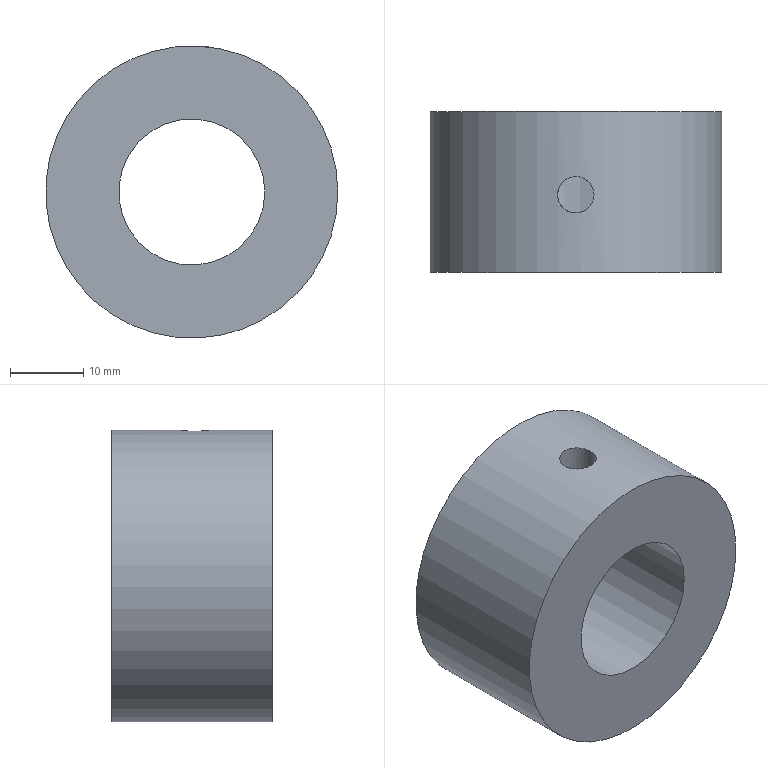Component | NX | BUSHING_5 | 1 solid | 5 faces | box 40 x 22 x 40 mm | volume 20537 mm3 | cylinder 3 | plane 2 | commonest cylinder face diameters 40 x1 20 x1 5 x1
STEP:
#1=CARTESIAN_POINT('',(0.,0.,0.));
#2=DIRECTION('',(0.,0.,1.));
#3=DIRECTION('',(1.,0.,0.));
#4=AXIS2_PLACEMENT_3D('',#1,#2,#3);
#5=CARTESIAN_POINT('',(1454.254,1145.,813.574));
#6=VERTEX_POINT('',#5);
#7=CARTESIAN_POINT('',(1434.254,1145.,813.574));
#8=DIRECTION('',(0.,1.,0.));
#9=DIRECTION('',(1.,0.,0.));
#10=AXIS2_PLACEMENT_3D('',#7,#8,#9);
#11=CIRCLE('',#10,20.);
#12=CARTESIAN_POINT('',(1434.254,1145.,813.574));
#13=DIRECTION('',(0.,-1.,0.));
#14=DIRECTION('',(0.,0.,-1.));
#15=AXIS2_PLACEMENT_3D('',#12,#13,#14);
#16=CYLINDRICAL_SURFACE('',#15,20.);
#17=CARTESIAN_POINT('',(7.854,0.));
#18=DIRECTION('',(-1.,0.));
#19=VECTOR('',#18,1.);
#20=LINE('',#17,#19);
#21=(GEOMETRIC_REPRESENTATION_CONTEXT(2)PARAMETRIC_REPRESENTATION_CONTEXT()REPRESENTATION_CONTEXT('',''));
#22=DEFINITIONAL_REPRESENTATION('',(#20),#21);
#23=PCURVE('',#16,#22);
#24=CARTESIAN_POINT('',(1434.254,1145.,813.574));
#25=DIRECTION('',(0.,1.,0.));
#26=DIRECTION('',(0.,0.,1.));
#27=AXIS2_PLACEMENT_3D('',#24,#25,#26);
#28=PLANE('',#27);
#29=CARTESIAN_POINT('',(0.,0.));
#30=DIRECTION('',(0.,1.));
#31=AXIS2_PLACEMENT_2D('',#29,#30);
#32=CIRCLE('',#31,20.);
#33=(GEOMETRIC_REPRESENTATION_CONTEXT(2)PARAMETRIC_REPRESENTATION_CONTEXT()REPRESENTATION_CONTEXT('',''));
#34=DEFINITIONAL_REPRESENTATION('',(#32),#33);
#35=PCURVE('',#28,#34);
#36=SURFACE_CURVE('',#11,(#23,#35),.PCURVE_S1.);
#37=EDGE_CURVE('',#6,#6,#36,.T.);
#38=ORIENTED_EDGE('',*,*,#37,.F.);
#39=CARTESIAN_POINT('',(1454.254,1123.,813.574));
#40=VERTEX_POINT('',#39);
#41=CARTESIAN_POINT('',(1454.254,1145.,813.574));
#42=CARTESIAN_POINT('',(1454.254,1123.,813.574));
#43=B_SPLINE_CURVE_WITH_KNOTS('',1,(#41,#42),.UNSPECIFIED.,.F.,.F.,(2,2),(0.,22.),.PIECEWISE_BEZIER_KNOTS.);
#44=CARTESIAN_POINT('',(7.854,0.));
#45=DIRECTION('',(0.,1.));
#46=VECTOR('',#45,1.);
#47=LINE('',#44,#46);
#48=(GEOMETRIC_REPRESENTATION_CONTEXT(2)PARAMETRIC_REPRESENTATION_CONTEXT()REPRESENTATION_CONTEXT('',''));
#49=DEFINITIONAL_REPRESENTATION('',(#47),#48);
#50=PCURVE('',#16,#49);
#51=CARTESIAN_POINT('',(1.571,0.));
#52=DIRECTION('',(0.,1.));
#53=VECTOR('',#52,1.);
#54=LINE('',#51,#53);
#55=(GEOMETRIC_REPRESENTATION_CONTEXT(2)PARAMETRIC_REPRESENTATION_CONTEXT()REPRESENTATION_CONTEXT('',''));
#56=DEFINITIONAL_REPRESENTATION('',(#54),#55);
#57=PCURVE('',#16,#56);
#58=SEAM_CURVE('',#43,(#50,#57),.PCURVE_S1.);
#59=EDGE_CURVE('',#6,#40,#58,.T.);
#60=ORIENTED_EDGE('',*,*,#59,.T.);
#61=CARTESIAN_POINT('',(1434.254,1123.,813.574));
#62=DIRECTION('',(0.,1.,0.));
#63=DIRECTION('',(1.,0.,0.));
#64=AXIS2_PLACEMENT_3D('',#61,#62,#63);
#65=CIRCLE('',#64,20.);
#66=CARTESIAN_POINT('',(7.854,22.));
#67=DIRECTION('',(-1.,0.));
#68=VECTOR('',#67,1.);
#69=LINE('',#66,#68);
#70=(GEOMETRIC_REPRESENTATION_CONTEXT(2)PARAMETRIC_REPRESENTATION_CONTEXT()REPRESENTATION_CONTEXT('',''));
#71=DEFINITIONAL_REPRESENTATION('',(#69),#70);
#72=PCURVE('',#16,#71);
#73=CARTESIAN_POINT('',(1434.254,1123.,813.574));
#74=DIRECTION('',(0.,1.,0.));
#75=DIRECTION('',(0.,0.,1.));
#76=AXIS2_PLACEMENT_3D('',#73,#74,#75);
#77=PLANE('',#76);
#78=CARTESIAN_POINT('',(0.,0.));
#79=DIRECTION('',(0.,1.));
#80=AXIS2_PLACEMENT_2D('',#78,#79);
#81=CIRCLE('',#80,20.);
#82=(GEOMETRIC_REPRESENTATION_CONTEXT(2)PARAMETRIC_REPRESENTATION_CONTEXT()REPRESENTATION_CONTEXT('',''));
#83=DEFINITIONAL_REPRESENTATION('',(#81),#82);
#84=PCURVE('',#77,#83);
#85=SURFACE_CURVE('',#65,(#72,#84),.PCURVE_S1.);
#86=EDGE_CURVE('',#40,#40,#85,.T.);
#87=ORIENTED_EDGE('',*,*,#86,.T.);
#88=ORIENTED_EDGE('',*,*,#59,.F.);
#89=EDGE_LOOP('',(#38,#60,#87,#88));
#90=FACE_BOUND('',#89,.T.);
#91=CARTESIAN_POINT('',(1436.754,1133.59,833.417));
#92=VERTEX_POINT('',#91);
#93=CARTESIAN_POINT('',(1436.754,1133.59,833.417));
#94=CARTESIAN_POINT('',(1436.754,1133.312,833.417));
#95=CARTESIAN_POINT('',(1436.706,1133.029,833.423));
#96=CARTESIAN_POINT('',(1436.615,1132.766,833.434));
#97=CARTESIAN_POINT('',(1436.523,1132.504,833.445));
#98=CARTESIAN_POINT('',(1436.385,1132.253,833.46));
#99=CARTESIAN_POINT('',(1436.212,1132.036,833.478));
#100=CARTESIAN_POINT('',(1436.038,1131.817,833.495));
#101=CARTESIAN_POINT('',(1435.824,1131.625,833.513));
#102=CARTESIAN_POINT('',(1435.588,1131.476,833.529));
#103=CARTESIAN_POINT('',(1435.351,1131.326,833.545));
#104=CARTESIAN_POINT('',(1435.084,1131.216,833.558));
#105=CARTESIAN_POINT('',(1434.811,1131.153,833.566));
#106=CARTESIAN_POINT('',(1434.539,1131.091,833.573));
#107=CARTESIAN_POINT('',(1434.252,1131.075,833.575));
#108=CARTESIAN_POINT('',(1433.974,1131.106,833.572));
#109=CARTESIAN_POINT('',(1433.698,1131.137,833.568));
#110=CARTESIAN_POINT('',(1433.424,1131.216,833.558));
#111=CARTESIAN_POINT('',(1433.173,1131.336,833.544));
#112=CARTESIAN_POINT('',(1432.923,1131.456,833.531));
#113=CARTESIAN_POINT('',(1432.689,1131.621,833.513));
#114=CARTESIAN_POINT('',(1432.492,1131.817,833.496));
#115=CARTESIAN_POINT('',(1432.293,1132.014,833.478));
#116=CARTESIAN_POINT('',(1432.126,1132.249,833.46));
#117=CARTESIAN_POINT('',(1432.004,1132.501,833.447));
#118=CARTESIAN_POINT('',(1431.882,1132.753,833.433));
#119=CARTESIAN_POINT('',(1431.802,1133.03,833.423));
#120=CARTESIAN_POINT('',(1431.77,1133.309,833.419));
#121=CARTESIAN_POINT('',(1431.739,1133.586,833.415));
#122=CARTESIAN_POINT('',(1431.754,1133.872,833.417));
#123=CARTESIAN_POINT('',(1431.816,1134.143,833.424));
#124=CARTESIAN_POINT('',(1431.878,1134.414,833.432));
#125=CARTESIAN_POINT('',(1431.986,1134.678,833.445));
#126=CARTESIAN_POINT('',(1432.133,1134.913,833.461));
#127=CARTESIAN_POINT('',(1432.28,1135.15,833.476));
#128=CARTESIAN_POINT('',(1432.47,1135.364,833.495));
#129=CARTESIAN_POINT('',(1432.688,1135.539,833.512));
#130=CARTESIAN_POINT('',(1432.906,1135.714,833.529));
#131=CARTESIAN_POINT('',(1433.158,1135.855,833.545));
#132=CARTESIAN_POINT('',(1433.423,1135.948,833.556));
#133=CARTESIAN_POINT('',(1433.687,1136.041,833.567));
#134=CARTESIAN_POINT('',(1433.97,1136.09,833.573));
#135=CARTESIAN_POINT('',(1434.25,1136.09,833.574));
#136=CARTESIAN_POINT('',(1434.528,1136.091,833.574));
#137=CARTESIAN_POINT('',(1434.81,1136.043,833.568));
#138=CARTESIAN_POINT('',(1435.073,1135.952,833.557));
#139=CARTESIAN_POINT('',(1435.336,1135.861,833.546));
#140=CARTESIAN_POINT('',(1435.586,1135.724,833.53));
#141=CARTESIAN_POINT('',(1435.804,1135.552,833.513));
#142=CARTESIAN_POINT('',(1436.023,1135.379,833.496));
#143=CARTESIAN_POINT('',(1436.215,1135.166,833.478));
#144=CARTESIAN_POINT('',(1436.365,1134.93,833.462));
#145=CARTESIAN_POINT('',(1436.515,1134.693,833.446));
#146=CARTESIAN_POINT('',(1436.627,1134.427,833.432));
#147=CARTESIAN_POINT('',(1436.69,1134.154,833.425));
#148=CARTESIAN_POINT('',(1436.732,1133.97,833.419));
#149=CARTESIAN_POINT('',(1436.754,1133.779,833.417));
#150=CARTESIAN_POINT('',(1436.754,1133.59,833.417));
#151=B_SPLINE_CURVE_WITH_KNOTS('',3,(#93,#94,#95,#96,#97,#98,#99,#100,#101,#102,#103,#104,#105,#106,#107,#108,#109,#110,#111,#112,#113,#114,#115,#116,#117,#118,#119,#120,#121,#122,#123,#124,#125,#126,#127,#128,#129,#130,#131,#132,#133,#134,#135,#136,#137,#138,#139,#140,#141,#142,#143,#144,#145,#146,#147,#148,#149,#150),.UNSPECIFIED.,.T.,.F.,(1,3,3,3,3,3,3,3,3,3,3,3,3,3,3,3,3,3,3,3,3,1),(-0.03595,0.,0.05342,0.1068,0.1605,0.2143,0.2679,0.3212,0.3746,0.4283,0.4821,0.5356,0.5888,0.6424,0.6962,0.7499,0.8032,0.8565,0.9102,0.964,1.,1.053),.UNSPECIFIED.);
#152=CARTESIAN_POINT('',(3.016,11.41));
#153=CARTESIAN_POINT('',(3.016,11.469));
#154=CARTESIAN_POINT('',(3.016,11.588));
#155=CARTESIAN_POINT('',(3.017,11.766));
#156=CARTESIAN_POINT('',(3.019,11.942));
#157=CARTESIAN_POINT('',(3.021,12.116));
#158=CARTESIAN_POINT('',(3.024,12.284));
#159=CARTESIAN_POINT('',(3.028,12.449));
#160=CARTESIAN_POINT('',(3.032,12.609));
#161=CARTESIAN_POINT('',(3.036,12.763));
#162=CARTESIAN_POINT('',(3.041,12.91));
#163=CARTESIAN_POINT('',(3.047,13.048));
#164=CARTESIAN_POINT('',(3.053,13.178));
#165=CARTESIAN_POINT('',(3.06,13.3));
#166=CARTESIAN_POINT('',(3.067,13.412));
#167=CARTESIAN_POINT('',(3.074,13.514));
#168=CARTESIAN_POINT('',(3.082,13.605));
#169=CARTESIAN_POINT('',(3.09,13.685));
#170=CARTESIAN_POINT('',(3.098,13.753));
#171=CARTESIAN_POINT('',(3.106,13.81));
#172=CARTESIAN_POINT('',(3.115,13.854));
#173=CARTESIAN_POINT('',(3.124,13.886));
#174=CARTESIAN_POINT('',(3.133,13.905));
#175=CARTESIAN_POINT('',(3.142,13.912));
#176=CARTESIAN_POINT('',(3.151,13.905));
#177=CARTESIAN_POINT('',(3.159,13.886));
#178=CARTESIAN_POINT('',(3.168,13.855));
#179=CARTESIAN_POINT('',(3.177,13.81));
#180=CARTESIAN_POINT('',(3.185,13.754));
#181=CARTESIAN_POINT('',(3.194,13.686));
#182=CARTESIAN_POINT('',(3.202,13.606));
#183=CARTESIAN_POINT('',(3.209,13.515));
#184=CARTESIAN_POINT('',(3.217,13.413));
#185=CARTESIAN_POINT('',(3.224,13.301));
#186=CARTESIAN_POINT('',(3.23,13.18));
#187=CARTESIAN_POINT('',(3.236,13.049));
#188=CARTESIAN_POINT('',(3.242,12.91));
#189=CARTESIAN_POINT('',(3.247,12.763));
#190=CARTESIAN_POINT('',(3.252,12.61));
#191=CARTESIAN_POINT('',(3.256,12.451));
#192=CARTESIAN_POINT('',(3.259,12.286));
#193=CARTESIAN_POINT('',(3.262,12.116));
#194=CARTESIAN_POINT('',(3.264,11.943));
#195=CARTESIAN_POINT('',(3.266,11.767));
#196=CARTESIAN_POINT('',(3.267,11.59));
#197=CARTESIAN_POINT('',(3.267,11.412));
#198=CARTESIAN_POINT('',(3.267,11.232));
#199=CARTESIAN_POINT('',(3.266,11.054));
#200=CARTESIAN_POINT('',(3.264,10.879));
#201=CARTESIAN_POINT('',(3.262,10.706));
#202=CARTESIAN_POINT('',(3.259,10.537));
#203=CARTESIAN_POINT('',(3.256,10.371));
#204=CARTESIAN_POINT('',(3.252,10.211));
#205=CARTESIAN_POINT('',(3.247,10.058));
#206=CARTESIAN_POINT('',(3.242,9.912));
#207=CARTESIAN_POINT('',(3.236,9.773));
#208=CARTESIAN_POINT('',(3.23,9.642));
#209=CARTESIAN_POINT('',(3.224,9.52));
#210=CARTESIAN_POINT('',(3.217,9.408));
#211=CARTESIAN_POINT('',(3.209,9.306));
#212=CARTESIAN_POINT('',(3.202,9.215));
#213=CARTESIAN_POINT('',(3.194,9.135));
#214=CARTESIAN_POINT('',(3.185,9.066));
#215=CARTESIAN_POINT('',(3.177,9.01));
#216=CARTESIAN_POINT('',(3.168,8.966));
#217=CARTESIAN_POINT('',(3.16,8.934));
#218=CARTESIAN_POINT('',(3.151,8.914));
#219=CARTESIAN_POINT('',(3.142,8.908));
#220=CARTESIAN_POINT('',(3.133,8.914));
#221=CARTESIAN_POINT('',(3.124,8.933));
#222=CARTESIAN_POINT('',(3.115,8.965));
#223=CARTESIAN_POINT('',(3.106,9.009));
#224=CARTESIAN_POINT('',(3.098,9.065));
#225=CARTESIAN_POINT('',(3.09,9.133));
#226=CARTESIAN_POINT('',(3.082,9.213));
#227=CARTESIAN_POINT('',(3.074,9.304));
#228=CARTESIAN_POINT('',(3.067,9.406));
#229=CARTESIAN_POINT('',(3.06,9.517));
#230=CARTESIAN_POINT('',(3.053,9.639));
#231=CARTESIAN_POINT('',(3.047,9.769));
#232=CARTESIAN_POINT('',(3.041,9.908));
#233=CARTESIAN_POINT('',(3.036,10.054));
#234=CARTESIAN_POINT('',(3.032,10.207));
#235=CARTESIAN_POINT('',(3.028,10.367));
#236=CARTESIAN_POINT('',(3.024,10.532));
#237=CARTESIAN_POINT('',(3.021,10.702));
#238=CARTESIAN_POINT('',(3.019,10.874));
#239=CARTESIAN_POINT('',(3.017,11.051));
#240=CARTESIAN_POINT('',(3.016,11.23));
#241=CARTESIAN_POINT('',(3.016,11.35));
#242=CARTESIAN_POINT('',(3.016,11.41));
#243=B_SPLINE_CURVE_WITH_KNOTS('',3,(#152,#153,#154,#155,#156,#157,#158,#159,#160,#161,#162,#163,#164,#165,#166,#167,#168,#169,#170,#171,#172,#173,#174,#175,#176,#177,#178,#179,#180,#181,#182,#183,#184,#185,#186,#187,#188,#189,#190,#191,#192,#193,#194,#195,#196,#197,#198,#199,#200,#201,#202,#203,#204,#205,#206,#207,#208,#209,#210,#211,#212,#213,#214,#215,#216,#217,#218,#219,#220,#221,#222,#223,#224,#225,#226,#227,#228,#229,#230,#231,#232,#233,#234,#235,#236,#237,#238,#239,#240,#241,#242),.UNSPECIFIED.,.T.,.F.,(4,1,1,1,1,1,1,1,1,1,1,1,1,1,1,1,1,1,1,1,1,1,1,1,1,1,1,1,1,1,1,1,1,1,1,1,1,1,1,1,1,1,1,1,1,1,1,1,1,1,1,1,1,1,1,1,1,1,1,1,1,1,1,1,1,1,1,1,1,1,1,1,1,1,1,1,1,1,1,1,1,1,1,1,1,1,1,1,4),(0.,0.01136,0.02273,0.03409,0.04545,0.05682,0.06818,0.07955,0.09091,0.1023,0.1136,0.125,0.1364,0.1477,0.1591,0.1705,0.1818,0.1932,0.2045,0.2159,0.2273,0.2386,0.25,0.2614,0.2727,0.2841,0.2955,0.3068,0.3182,0.3295,0.3409,0.3523,0.3636,0.375,0.3864,0.3977,0.4091,0.4205,0.4318,0.4432,0.4545,0.4659,0.4773,0.4886,0.5,0.5114,0.5227,0.5341,0.5455,0.5568,0.5682,0.5795,0.5909,0.6023,0.6136,0.625,0.6364,0.6477,0.6591,0.6705,0.6818,0.6932,0.7045,0.7159,0.7273,0.7386,0.75,0.7614,0.7727,0.7841,0.7955,0.8068,0.8182,0.8295,0.8409,0.8523,0.8636,0.875,0.8864,0.8977,0.9091,0.9205,0.9318,0.9432,0.9545,0.9659,0.9773,0.9886,1.),.QUASI_UNIFORM_KNOTS.);
#244=(GEOMETRIC_REPRESENTATION_CONTEXT(2)PARAMETRIC_REPRESENTATION_CONTEXT()REPRESENTATION_CONTEXT('',''));
#245=DEFINITIONAL_REPRESENTATION('',(#243),#244);
#246=PCURVE('',#16,#245);
#247=CARTESIAN_POINT('',(1434.254,1133.59,813.574));
#248=DIRECTION('',(-0.,0.,1.));
#249=DIRECTION('',(1.,0.,0.));
#250=AXIS2_PLACEMENT_3D('',#247,#248,#249);
#251=CYLINDRICAL_SURFACE('',#250,2.5);
#252=CARTESIAN_POINT('',(6.283,19.843));
#253=CARTESIAN_POINT('',(6.259,19.843));
#254=CARTESIAN_POINT('',(6.212,19.844));
#255=CARTESIAN_POINT('',(6.14,19.846));
#256=CARTESIAN_POINT('',(6.069,19.85));
#257=CARTESIAN_POINT('',(5.997,19.855));
#258=CARTESIAN_POINT('',(5.926,19.862));
#259=CARTESIAN_POINT('',(5.855,19.87));
#260=CARTESIAN_POINT('',(5.783,19.879));
#261=CARTESIAN_POINT('',(5.712,19.889));
#262=CARTESIAN_POINT('',(5.64,19.9));
#263=CARTESIAN_POINT('',(5.569,19.91));
#264=CARTESIAN_POINT('',(5.498,19.922));
#265=CARTESIAN_POINT('',(5.427,19.933));
#266=CARTESIAN_POINT('',(5.355,19.944));
#267=CARTESIAN_POINT('',(5.284,19.954));
#268=CARTESIAN_POINT('',(5.213,19.964));
#269=CARTESIAN_POINT('',(5.141,19.973));
#270=CARTESIAN_POINT('',(5.07,19.981));
#271=CARTESIAN_POINT('',(4.998,19.988));
#272=CARTESIAN_POINT('',(4.927,19.993));
#273=CARTESIAN_POINT('',(4.856,19.997));
#274=CARTESIAN_POINT('',(4.784,19.999));
#275=CARTESIAN_POINT('',(4.713,20.));
#276=CARTESIAN_POINT('',(4.641,19.999));
#277=CARTESIAN_POINT('',(4.57,19.997));
#278=CARTESIAN_POINT('',(4.499,19.993));
#279=CARTESIAN_POINT('',(4.427,19.988));
#280=CARTESIAN_POINT('',(4.355,19.981));
#281=CARTESIAN_POINT('',(4.284,19.973));
#282=CARTESIAN_POINT('',(4.213,19.964));
#283=CARTESIAN_POINT('',(4.142,19.954));
#284=CARTESIAN_POINT('',(4.07,19.944));
#285=CARTESIAN_POINT('',(3.999,19.933));
#286=CARTESIAN_POINT('',(3.927,19.922));
#287=CARTESIAN_POINT('',(3.856,19.911));
#288=CARTESIAN_POINT('',(3.785,19.9));
#289=CARTESIAN_POINT('',(3.713,19.889));
#290=CARTESIAN_POINT('',(3.642,19.879));
#291=CARTESIAN_POINT('',(3.571,19.87));
#292=CARTESIAN_POINT('',(3.5,19.862));
#293=CARTESIAN_POINT('',(3.428,19.856));
#294=CARTESIAN_POINT('',(3.356,19.85));
#295=CARTESIAN_POINT('',(3.285,19.846));
#296=CARTESIAN_POINT('',(3.214,19.844));
#297=CARTESIAN_POINT('',(3.142,19.843));
#298=CARTESIAN_POINT('',(3.071,19.844));
#299=CARTESIAN_POINT('',(2.999,19.846));
#300=CARTESIAN_POINT('',(2.928,19.85));
#301=CARTESIAN_POINT('',(2.857,19.855));
#302=CARTESIAN_POINT('',(2.785,19.862));
#303=CARTESIAN_POINT('',(2.714,19.87));
#304=CARTESIAN_POINT('',(2.642,19.879));
#305=CARTESIAN_POINT('',(2.571,19.889));
#306=CARTESIAN_POINT('',(2.5,19.899));
#307=CARTESIAN_POINT('',(2.428,19.91));
#308=CARTESIAN_POINT('',(2.357,19.922));
#309=CARTESIAN_POINT('',(2.285,19.933));
#310=CARTESIAN_POINT('',(2.214,19.944));
#311=CARTESIAN_POINT('',(2.143,19.954));
#312=CARTESIAN_POINT('',(2.072,19.964));
#313=CARTESIAN_POINT('',(2.,19.973));
#314=CARTESIAN_POINT('',(1.929,19.981));
#315=CARTESIAN_POINT('',(1.858,19.988));
#316=CARTESIAN_POINT('',(1.786,19.993));
#317=CARTESIAN_POINT('',(1.715,19.997));
#318=CARTESIAN_POINT('',(1.643,19.999));
#319=CARTESIAN_POINT('',(1.572,20.));
#320=CARTESIAN_POINT('',(1.5,19.999));
#321=CARTESIAN_POINT('',(1.429,19.997));
#322=CARTESIAN_POINT('',(1.357,19.993));
#323=CARTESIAN_POINT('',(1.286,19.988));
#324=CARTESIAN_POINT('',(1.215,19.981));
#325=CARTESIAN_POINT('',(1.143,19.973));
#326=CARTESIAN_POINT('',(1.072,19.964));
#327=CARTESIAN_POINT('',(1.,19.954));
#328=CARTESIAN_POINT('',(0.9289,19.944));
#329=CARTESIAN_POINT('',(0.8579,19.933));
#330=CARTESIAN_POINT('',(0.7865,19.922));
#331=CARTESIAN_POINT('',(0.715,19.911));
#332=CARTESIAN_POINT('',(0.6436,19.9));
#333=CARTESIAN_POINT('',(0.5724,19.889));
#334=CARTESIAN_POINT('',(0.5013,19.879));
#335=CARTESIAN_POINT('',(0.4298,19.87));
#336=CARTESIAN_POINT('',(0.3582,19.862));
#337=CARTESIAN_POINT('',(0.2867,19.856));
#338=CARTESIAN_POINT('',(0.2156,19.85));
#339=CARTESIAN_POINT('',(0.1437,19.846));
#340=CARTESIAN_POINT('',(0.07178,19.844));
#341=CARTESIAN_POINT('',(0.02389,19.843));
#342=CARTESIAN_POINT('',(0.,19.843));
#343=B_SPLINE_CURVE_WITH_KNOTS('',3,(#252,#253,#254,#255,#256,#257,#258,#259,#260,#261,#262,#263,#264,#265,#266,#267,#268,#269,#270,#271,#272,#273,#274,#275,#276,#277,#278,#279,#280,#281,#282,#283,#284,#285,#286,#287,#288,#289,#290,#291,#292,#293,#294,#295,#296,#297,#298,#299,#300,#301,#302,#303,#304,#305,#306,#307,#308,#309,#310,#311,#312,#313,#314,#315,#316,#317,#318,#319,#320,#321,#322,#323,#324,#325,#326,#327,#328,#329,#330,#331,#332,#333,#334,#335,#336,#337,#338,#339,#340,#341,#342),.UNSPECIFIED.,.F.,.F.,(4,1,1,1,1,1,1,1,1,1,1,1,1,1,1,1,1,1,1,1,1,1,1,1,1,1,1,1,1,1,1,1,1,1,1,1,1,1,1,1,1,1,1,1,1,1,1,1,1,1,1,1,1,1,1,1,1,1,1,1,1,1,1,1,1,1,1,1,1,1,1,1,1,1,1,1,1,1,1,1,1,1,1,1,1,1,1,1,4),(0.,0.01136,0.02273,0.03409,0.04545,0.05682,0.06818,0.07955,0.09091,0.1023,0.1136,0.125,0.1364,0.1477,0.1591,0.1705,0.1818,0.1932,0.2045,0.2159,0.2273,0.2386,0.25,0.2614,0.2727,0.2841,0.2955,0.3068,0.3182,0.3295,0.3409,0.3523,0.3636,0.375,0.3864,0.3977,0.4091,0.4205,0.4318,0.4432,0.4545,0.4659,0.4773,0.4886,0.5,0.5114,0.5227,0.5341,0.5455,0.5568,0.5682,0.5795,0.5909,0.6023,0.6136,0.625,0.6364,0.6477,0.6591,0.6705,0.6818,0.6932,0.7045,0.7159,0.7273,0.7386,0.75,0.7614,0.7727,0.7841,0.7955,0.8068,0.8182,0.8295,0.8409,0.8523,0.8636,0.875,0.8864,0.8977,0.9091,0.9205,0.9318,0.9432,0.9545,0.9659,0.9773,0.9886,1.),.QUASI_UNIFORM_KNOTS.);
#344=(GEOMETRIC_REPRESENTATION_CONTEXT(2)PARAMETRIC_REPRESENTATION_CONTEXT()REPRESENTATION_CONTEXT('',''));
#345=DEFINITIONAL_REPRESENTATION('',(#343),#344);
#346=PCURVE('',#251,#345);
#347=SURFACE_CURVE('',#151,(#246,#346),.PCURVE_S1.);
#348=EDGE_CURVE('',#92,#92,#347,.T.);
#349=ORIENTED_EDGE('',*,*,#348,.T.);
#350=EDGE_LOOP('',(#349));
#351=FACE_BOUND('',#350,.T.);
#352=ADVANCED_FACE('',(#90,#351),#16,.T.);
#353=CARTESIAN_POINT('',(1444.254,1145.,813.574));
#354=VERTEX_POINT('',#353);
#355=CARTESIAN_POINT('',(1434.254,1145.,813.574));
#356=DIRECTION('',(0.,1.,0.));
#357=DIRECTION('',(1.,0.,0.));
#358=AXIS2_PLACEMENT_3D('',#355,#356,#357);
#359=CIRCLE('',#358,10.);
#360=CARTESIAN_POINT('',(1434.254,1145.,813.574));
#361=DIRECTION('',(0.,-1.,0.));
#362=DIRECTION('',(0.,0.,-1.));
#363=AXIS2_PLACEMENT_3D('',#360,#361,#362);
#364=CYLINDRICAL_SURFACE('',#363,10.);
#365=CARTESIAN_POINT('',(7.854,0.));
#366=DIRECTION('',(-1.,0.));
#367=VECTOR('',#366,1.);
#368=LINE('',#365,#367);
#369=(GEOMETRIC_REPRESENTATION_CONTEXT(2)PARAMETRIC_REPRESENTATION_CONTEXT()REPRESENTATION_CONTEXT('',''));
#370=DEFINITIONAL_REPRESENTATION('',(#368),#369);
#371=PCURVE('',#364,#370);
#372=CARTESIAN_POINT('',(0.,0.));
#373=DIRECTION('',(0.,1.));
#374=AXIS2_PLACEMENT_2D('',#372,#373);
#375=CIRCLE('',#374,10.);
#376=(GEOMETRIC_REPRESENTATION_CONTEXT(2)PARAMETRIC_REPRESENTATION_CONTEXT()REPRESENTATION_CONTEXT('',''));
#377=DEFINITIONAL_REPRESENTATION('',(#375),#376);
#378=PCURVE('',#28,#377);
#379=SURFACE_CURVE('',#359,(#371,#378),.PCURVE_S1.);
#380=EDGE_CURVE('',#354,#354,#379,.T.);
#381=ORIENTED_EDGE('',*,*,#380,.F.);
#382=CARTESIAN_POINT('',(1444.254,1123.,813.574));
#383=VERTEX_POINT('',#382);
#384=CARTESIAN_POINT('',(1444.254,1145.,813.574));
#385=CARTESIAN_POINT('',(1444.254,1123.,813.574));
#386=B_SPLINE_CURVE_WITH_KNOTS('',1,(#384,#385),.UNSPECIFIED.,.F.,.F.,(2,2),(0.,22.),.PIECEWISE_BEZIER_KNOTS.);
#387=CARTESIAN_POINT('',(7.854,0.));
#388=DIRECTION('',(0.,1.));
#389=VECTOR('',#388,1.);
#390=LINE('',#387,#389);
#391=(GEOMETRIC_REPRESENTATION_CONTEXT(2)PARAMETRIC_REPRESENTATION_CONTEXT()REPRESENTATION_CONTEXT('',''));
#392=DEFINITIONAL_REPRESENTATION('',(#390),#391);
#393=PCURVE('',#364,#392);
#394=CARTESIAN_POINT('',(1.571,0.));
#395=DIRECTION('',(0.,1.));
#396=VECTOR('',#395,1.);
#397=LINE('',#394,#396);
#398=(GEOMETRIC_REPRESENTATION_CONTEXT(2)PARAMETRIC_REPRESENTATION_CONTEXT()REPRESENTATION_CONTEXT('',''));
#399=DEFINITIONAL_REPRESENTATION('',(#397),#398);
#400=PCURVE('',#364,#399);
#401=SEAM_CURVE('',#386,(#393,#400),.PCURVE_S1.);
#402=EDGE_CURVE('',#354,#383,#401,.T.);
#403=ORIENTED_EDGE('',*,*,#402,.T.);
#404=CARTESIAN_POINT('',(1434.254,1123.,813.574));
#405=DIRECTION('',(0.,1.,0.));
#406=DIRECTION('',(1.,0.,0.));
#407=AXIS2_PLACEMENT_3D('',#404,#405,#406);
#408=CIRCLE('',#407,10.);
#409=CARTESIAN_POINT('',(7.854,22.));
#410=DIRECTION('',(-1.,0.));
#411=VECTOR('',#410,1.);
#412=LINE('',#409,#411);
#413=(GEOMETRIC_REPRESENTATION_CONTEXT(2)PARAMETRIC_REPRESENTATION_CONTEXT()REPRESENTATION_CONTEXT('',''));
#414=DEFINITIONAL_REPRESENTATION('',(#412),#413);
#415=PCURVE('',#364,#414);
#416=CARTESIAN_POINT('',(0.,0.));
#417=DIRECTION('',(0.,1.));
#418=AXIS2_PLACEMENT_2D('',#416,#417);
#419=CIRCLE('',#418,10.);
#420=(GEOMETRIC_REPRESENTATION_CONTEXT(2)PARAMETRIC_REPRESENTATION_CONTEXT()REPRESENTATION_CONTEXT('',''));
#421=DEFINITIONAL_REPRESENTATION('',(#419),#420);
#422=PCURVE('',#77,#421);
#423=SURFACE_CURVE('',#408,(#415,#422),.PCURVE_S1.);
#424=EDGE_CURVE('',#383,#383,#423,.T.);
#425=ORIENTED_EDGE('',*,*,#424,.T.);
#426=ORIENTED_EDGE('',*,*,#402,.F.);
#427=EDGE_LOOP('',(#381,#403,#425,#426));
#428=FACE_BOUND('',#427,.F.);
#429=CARTESIAN_POINT('',(1436.754,1133.59,823.256));
#430=VERTEX_POINT('',#429);
#431=CARTESIAN_POINT('',(1436.754,1133.59,823.256));
#432=CARTESIAN_POINT('',(1436.754,1133.315,823.256));
#433=CARTESIAN_POINT('',(1436.707,1133.037,823.268));
#434=CARTESIAN_POINT('',(1436.618,1132.778,823.29));
#435=CARTESIAN_POINT('',(1436.529,1132.519,823.312));
#436=CARTESIAN_POINT('',(1436.396,1132.272,823.343));
#437=CARTESIAN_POINT('',(1436.229,1132.057,823.377));
#438=CARTESIAN_POINT('',(1436.058,1131.837,823.411));
#439=CARTESIAN_POINT('',(1435.848,1131.644,823.449));
#440=CARTESIAN_POINT('',(1435.614,1131.493,823.481));
#441=CARTESIAN_POINT('',(1435.378,1131.339,823.513));
#442=CARTESIAN_POINT('',(1435.11,1131.224,823.541));
#443=CARTESIAN_POINT('',(1434.834,1131.159,823.557));
#444=CARTESIAN_POINT('',(1434.564,1131.094,823.572));
#445=CARTESIAN_POINT('',(1434.278,1131.075,823.577));
#446=CARTESIAN_POINT('',(1434.002,1131.103,823.57));
#447=CARTESIAN_POINT('',(1433.731,1131.131,823.564));
#448=CARTESIAN_POINT('',(1433.462,1131.204,823.545));
#449=CARTESIAN_POINT('',(1433.216,1131.316,823.519));
#450=CARTESIAN_POINT('',(1432.967,1131.43,823.494));
#451=CARTESIAN_POINT('',(1432.735,1131.586,823.459));
#452=CARTESIAN_POINT('',(1432.537,1131.774,823.425));
#453=CARTESIAN_POINT('',(1432.334,1131.966,823.39));
#454=CARTESIAN_POINT('',(1432.161,1132.195,823.353));
#455=CARTESIAN_POINT('',(1432.032,1132.445,823.324));
#456=CARTESIAN_POINT('',(1431.903,1132.695,823.294));
#457=CARTESIAN_POINT('',(1431.815,1132.973,823.272));
#458=CARTESIAN_POINT('',(1431.777,1133.253,823.262));
#459=CARTESIAN_POINT('',(1431.74,1133.526,823.252));
#460=CARTESIAN_POINT('',(1431.749,1133.81,823.255));
#461=CARTESIAN_POINT('',(1431.803,1134.08,823.268));
#462=CARTESIAN_POINT('',(1431.856,1134.346,823.282));
#463=CARTESIAN_POINT('',(1431.954,1134.605,823.306));
#464=CARTESIAN_POINT('',(1432.088,1134.839,823.336));
#465=CARTESIAN_POINT('',(1432.226,1135.077,823.367));
#466=CARTESIAN_POINT('',(1432.405,1135.295,823.403));
#467=CARTESIAN_POINT('',(1432.612,1135.475,823.438));
#468=CARTESIAN_POINT('',(1432.824,1135.66,823.473));
#469=CARTESIAN_POINT('',(1433.072,1135.811,823.507));
#470=CARTESIAN_POINT('',(1433.334,1135.915,823.531));
#471=CARTESIAN_POINT('',(1433.595,1136.018,823.555));
#472=CARTESIAN_POINT('',(1433.878,1136.078,823.57));
#473=CARTESIAN_POINT('',(1434.159,1136.089,823.573));
#474=CARTESIAN_POINT('',(1434.433,1136.099,823.576));
#475=CARTESIAN_POINT('',(1434.712,1136.063,823.566));
#476=CARTESIAN_POINT('',(1434.974,1135.984,823.548));
#477=CARTESIAN_POINT('',(1435.234,1135.906,823.529));
#478=CARTESIAN_POINT('',(1435.484,1135.784,823.5));
#479=CARTESIAN_POINT('',(1435.704,1135.627,823.468));
#480=CARTESIAN_POINT('',(1435.93,1135.466,823.435));
#481=CARTESIAN_POINT('',(1436.131,1135.265,823.397));
#482=CARTESIAN_POINT('',(1436.291,1135.039,823.364));
#483=CARTESIAN_POINT('',(1436.455,1134.81,823.33));
#484=CARTESIAN_POINT('',(1436.581,1134.547,823.299));
#485=CARTESIAN_POINT('',(1436.659,1134.275,823.28));
#486=CARTESIAN_POINT('',(1436.722,1134.054,823.265));
#487=CARTESIAN_POINT('',(1436.754,1133.821,823.256));
#488=CARTESIAN_POINT('',(1436.754,1133.59,823.256));
#489=B_SPLINE_CURVE_WITH_KNOTS('',3,(#431,#432,#433,#434,#435,#436,#437,#438,#439,#440,#441,#442,#443,#444,#445,#446,#447,#448,#449,#450,#451,#452,#453,#454,#455,#456,#457,#458,#459,#460,#461,#462,#463,#464,#465,#466,#467,#468,#469,#470,#471,#472,#473,#474,#475,#476,#477,#478,#479,#480,#481,#482,#483,#484,#485,#486,#487,#488),.UNSPECIFIED.,.T.,.F.,(1,3,3,3,3,3,3,3,3,3,3,3,3,3,3,3,3,3,3,3,3,1),(-0.04388,0.,0.05255,0.105,0.1586,0.2129,0.2661,0.3181,0.3705,0.4244,0.4786,0.5314,0.5832,0.6361,0.6903,0.7441,0.7964,0.8485,0.9018,0.9561,1.,1.053),.UNSPECIFIED.);
#490=CARTESIAN_POINT('',(2.889,11.41));
#491=CARTESIAN_POINT('',(2.889,11.469));
#492=CARTESIAN_POINT('',(2.889,11.588));
#493=CARTESIAN_POINT('',(2.891,11.767));
#494=CARTESIAN_POINT('',(2.895,11.944));
#495=CARTESIAN_POINT('',(2.899,12.117));
#496=CARTESIAN_POINT('',(2.905,12.286));
#497=CARTESIAN_POINT('',(2.912,12.451));
#498=CARTESIAN_POINT('',(2.92,12.611));
#499=CARTESIAN_POINT('',(2.93,12.764));
#500=CARTESIAN_POINT('',(2.94,12.91));
#501=CARTESIAN_POINT('',(2.951,13.048));
#502=CARTESIAN_POINT('',(2.964,13.178));
#503=CARTESIAN_POINT('',(2.977,13.3));
#504=CARTESIAN_POINT('',(2.991,13.412));
#505=CARTESIAN_POINT('',(3.006,13.513));
#506=CARTESIAN_POINT('',(3.021,13.604));
#507=CARTESIAN_POINT('',(3.037,13.684));
#508=CARTESIAN_POINT('',(3.054,13.753));
#509=CARTESIAN_POINT('',(3.071,13.81));
#510=CARTESIAN_POINT('',(3.088,13.854));
#511=CARTESIAN_POINT('',(3.106,13.886));
#512=CARTESIAN_POINT('',(3.124,13.905));
#513=CARTESIAN_POINT('',(3.142,13.912));
#514=CARTESIAN_POINT('',(3.159,13.905));
#515=CARTESIAN_POINT('',(3.177,13.886));
#516=CARTESIAN_POINT('',(3.195,13.854));
#517=CARTESIAN_POINT('',(3.212,13.81));
#518=CARTESIAN_POINT('',(3.229,13.753));
#519=CARTESIAN_POINT('',(3.246,13.685));
#520=CARTESIAN_POINT('',(3.262,13.605));
#521=CARTESIAN_POINT('',(3.277,13.514));
#522=CARTESIAN_POINT('',(3.292,13.412));
#523=CARTESIAN_POINT('',(3.306,13.3));
#524=CARTESIAN_POINT('',(3.319,13.18));
#525=CARTESIAN_POINT('',(3.332,13.049));
#526=CARTESIAN_POINT('',(3.343,12.911));
#527=CARTESIAN_POINT('',(3.354,12.764));
#528=CARTESIAN_POINT('',(3.363,12.611));
#529=CARTESIAN_POINT('',(3.371,12.453));
#530=CARTESIAN_POINT('',(3.378,12.288));
#531=CARTESIAN_POINT('',(3.384,12.118));
#532=CARTESIAN_POINT('',(3.389,11.944));
#533=CARTESIAN_POINT('',(3.392,11.768));
#534=CARTESIAN_POINT('',(3.394,11.591));
#535=CARTESIAN_POINT('',(3.394,11.411));
#536=CARTESIAN_POINT('',(3.394,11.232));
#537=CARTESIAN_POINT('',(3.392,11.053));
#538=CARTESIAN_POINT('',(3.389,10.878));
#539=CARTESIAN_POINT('',(3.384,10.704));
#540=CARTESIAN_POINT('',(3.378,10.534));
#541=CARTESIAN_POINT('',(3.371,10.369));
#542=CARTESIAN_POINT('',(3.363,10.209));
#543=CARTESIAN_POINT('',(3.354,10.057));
#544=CARTESIAN_POINT('',(3.343,9.911));
#545=CARTESIAN_POINT('',(3.332,9.772));
#546=CARTESIAN_POINT('',(3.319,9.641));
#547=CARTESIAN_POINT('',(3.306,9.52));
#548=CARTESIAN_POINT('',(3.292,9.409));
#549=CARTESIAN_POINT('',(3.278,9.307));
#550=CARTESIAN_POINT('',(3.262,9.215));
#551=CARTESIAN_POINT('',(3.246,9.135));
#552=CARTESIAN_POINT('',(3.23,9.067));
#553=CARTESIAN_POINT('',(3.213,9.01));
#554=CARTESIAN_POINT('',(3.195,8.966));
#555=CARTESIAN_POINT('',(3.177,8.934));
#556=CARTESIAN_POINT('',(3.16,8.914));
#557=CARTESIAN_POINT('',(3.142,8.908));
#558=CARTESIAN_POINT('',(3.124,8.914));
#559=CARTESIAN_POINT('',(3.106,8.933));
#560=CARTESIAN_POINT('',(3.088,8.965));
#561=CARTESIAN_POINT('',(3.071,9.009));
#562=CARTESIAN_POINT('',(3.054,9.065));
#563=CARTESIAN_POINT('',(3.037,9.134));
#564=CARTESIAN_POINT('',(3.021,9.214));
#565=CARTESIAN_POINT('',(3.006,9.305));
#566=CARTESIAN_POINT('',(2.991,9.406));
#567=CARTESIAN_POINT('',(2.977,9.518));
#568=CARTESIAN_POINT('',(2.964,9.64));
#569=CARTESIAN_POINT('',(2.951,9.77));
#570=CARTESIAN_POINT('',(2.94,9.908));
#571=CARTESIAN_POINT('',(2.93,10.054));
#572=CARTESIAN_POINT('',(2.92,10.207));
#573=CARTESIAN_POINT('',(2.912,10.367));
#574=CARTESIAN_POINT('',(2.905,10.532));
#575=CARTESIAN_POINT('',(2.899,10.701));
#576=CARTESIAN_POINT('',(2.895,10.874));
#577=CARTESIAN_POINT('',(2.891,11.051));
#578=CARTESIAN_POINT('',(2.889,11.23));
#579=CARTESIAN_POINT('',(2.889,11.35));
#580=CARTESIAN_POINT('',(2.889,11.41));
#581=B_SPLINE_CURVE_WITH_KNOTS('',3,(#490,#491,#492,#493,#494,#495,#496,#497,#498,#499,#500,#501,#502,#503,#504,#505,#506,#507,#508,#509,#510,#511,#512,#513,#514,#515,#516,#517,#518,#519,#520,#521,#522,#523,#524,#525,#526,#527,#528,#529,#530,#531,#532,#533,#534,#535,#536,#537,#538,#539,#540,#541,#542,#543,#544,#545,#546,#547,#548,#549,#550,#551,#552,#553,#554,#555,#556,#557,#558,#559,#560,#561,#562,#563,#564,#565,#566,#567,#568,#569,#570,#571,#572,#573,#574,#575,#576,#577,#578,#579,#580),.UNSPECIFIED.,.T.,.F.,(4,1,1,1,1,1,1,1,1,1,1,1,1,1,1,1,1,1,1,1,1,1,1,1,1,1,1,1,1,1,1,1,1,1,1,1,1,1,1,1,1,1,1,1,1,1,1,1,1,1,1,1,1,1,1,1,1,1,1,1,1,1,1,1,1,1,1,1,1,1,1,1,1,1,1,1,1,1,1,1,1,1,1,1,1,1,1,1,4),(0.,0.01136,0.02273,0.03409,0.04545,0.05682,0.06818,0.07955,0.09091,0.1023,0.1136,0.125,0.1364,0.1477,0.1591,0.1705,0.1818,0.1932,0.2045,0.2159,0.2273,0.2386,0.25,0.2614,0.2727,0.2841,0.2955,0.3068,0.3182,0.3295,0.3409,0.3523,0.3636,0.375,0.3864,0.3977,0.4091,0.4205,0.4318,0.4432,0.4545,0.4659,0.4773,0.4886,0.5,0.5114,0.5227,0.5341,0.5455,0.5568,0.5682,0.5795,0.5909,0.6023,0.6136,0.625,0.6364,0.6477,0.6591,0.6705,0.6818,0.6932,0.7045,0.7159,0.7273,0.7386,0.75,0.7614,0.7727,0.7841,0.7955,0.8068,0.8182,0.8295,0.8409,0.8523,0.8636,0.875,0.8864,0.8977,0.9091,0.9205,0.9318,0.9432,0.9545,0.9659,0.9773,0.9886,1.),.QUASI_UNIFORM_KNOTS.);
#582=(GEOMETRIC_REPRESENTATION_CONTEXT(2)PARAMETRIC_REPRESENTATION_CONTEXT()REPRESENTATION_CONTEXT('',''));
#583=DEFINITIONAL_REPRESENTATION('',(#581),#582);
#584=PCURVE('',#364,#583);
#585=CARTESIAN_POINT('',(6.283,9.682));
#586=CARTESIAN_POINT('',(6.259,9.682));
#587=CARTESIAN_POINT('',(6.212,9.684));
#588=CARTESIAN_POINT('',(6.14,9.689));
#589=CARTESIAN_POINT('',(6.068,9.697));
#590=CARTESIAN_POINT('',(5.997,9.708));
#591=CARTESIAN_POINT('',(5.925,9.722));
#592=CARTESIAN_POINT('',(5.854,9.738));
#593=CARTESIAN_POINT('',(5.783,9.756));
#594=CARTESIAN_POINT('',(5.711,9.776));
#595=CARTESIAN_POINT('',(5.64,9.798));
#596=CARTESIAN_POINT('',(5.569,9.82));
#597=CARTESIAN_POINT('',(5.498,9.842));
#598=CARTESIAN_POINT('',(5.427,9.865));
#599=CARTESIAN_POINT('',(5.355,9.887));
#600=CARTESIAN_POINT('',(5.284,9.908));
#601=CARTESIAN_POINT('',(5.213,9.928));
#602=CARTESIAN_POINT('',(5.142,9.946));
#603=CARTESIAN_POINT('',(5.07,9.962));
#604=CARTESIAN_POINT('',(4.999,9.975));
#605=CARTESIAN_POINT('',(4.928,9.986));
#606=CARTESIAN_POINT('',(4.856,9.994));
#607=CARTESIAN_POINT('',(4.784,9.999));
#608=CARTESIAN_POINT('',(4.713,10.));
#609=CARTESIAN_POINT('',(4.641,9.999));
#610=CARTESIAN_POINT('',(4.57,9.994));
#611=CARTESIAN_POINT('',(4.498,9.986));
#612=CARTESIAN_POINT('',(4.426,9.975));
#613=CARTESIAN_POINT('',(4.355,9.962));
#614=CARTESIAN_POINT('',(4.283,9.946));
#615=CARTESIAN_POINT('',(4.212,9.928));
#616=CARTESIAN_POINT('',(4.141,9.908));
#617=CARTESIAN_POINT('',(4.069,9.887));
#618=CARTESIAN_POINT('',(3.998,9.865));
#619=CARTESIAN_POINT('',(3.927,9.843));
#620=CARTESIAN_POINT('',(3.856,9.82));
#621=CARTESIAN_POINT('',(3.785,9.798));
#622=CARTESIAN_POINT('',(3.714,9.776));
#623=CARTESIAN_POINT('',(3.642,9.756));
#624=CARTESIAN_POINT('',(3.572,9.738));
#625=CARTESIAN_POINT('',(3.5,9.722));
#626=CARTESIAN_POINT('',(3.428,9.708));
#627=CARTESIAN_POINT('',(3.357,9.697));
#628=CARTESIAN_POINT('',(3.285,9.689));
#629=CARTESIAN_POINT('',(3.214,9.684));
#630=CARTESIAN_POINT('',(3.142,9.682));
#631=CARTESIAN_POINT('',(3.07,9.684));
#632=CARTESIAN_POINT('',(2.999,9.689));
#633=CARTESIAN_POINT('',(2.927,9.697));
#634=CARTESIAN_POINT('',(2.856,9.708));
#635=CARTESIAN_POINT('',(2.784,9.722));
#636=CARTESIAN_POINT('',(2.713,9.738));
#637=CARTESIAN_POINT('',(2.641,9.756));
#638=CARTESIAN_POINT('',(2.57,9.776));
#639=CARTESIAN_POINT('',(2.499,9.798));
#640=CARTESIAN_POINT('',(2.428,9.82));
#641=CARTESIAN_POINT('',(2.357,9.842));
#642=CARTESIAN_POINT('',(2.286,9.865));
#643=CARTESIAN_POINT('',(2.215,9.887));
#644=CARTESIAN_POINT('',(2.143,9.908));
#645=CARTESIAN_POINT('',(2.072,9.928));
#646=CARTESIAN_POINT('',(2.001,9.946));
#647=CARTESIAN_POINT('',(1.93,9.962));
#648=CARTESIAN_POINT('',(1.858,9.975));
#649=CARTESIAN_POINT('',(1.786,9.986));
#650=CARTESIAN_POINT('',(1.715,9.994));
#651=CARTESIAN_POINT('',(1.643,9.999));
#652=CARTESIAN_POINT('',(1.572,10.001));
#653=CARTESIAN_POINT('',(1.5,9.999));
#654=CARTESIAN_POINT('',(1.428,9.994));
#655=CARTESIAN_POINT('',(1.356,9.986));
#656=CARTESIAN_POINT('',(1.285,9.976));
#657=CARTESIAN_POINT('',(1.214,9.962));
#658=CARTESIAN_POINT('',(1.142,9.946));
#659=CARTESIAN_POINT('',(1.071,9.928));
#660=CARTESIAN_POINT('',(0.9993,9.908));
#661=CARTESIAN_POINT('',(0.9284,9.887));
#662=CARTESIAN_POINT('',(0.8573,9.865));
#663=CARTESIAN_POINT('',(0.786,9.843));
#664=CARTESIAN_POINT('',(0.7147,9.82));
#665=CARTESIAN_POINT('',(0.6436,9.798));
#666=CARTESIAN_POINT('',(0.5728,9.777));
#667=CARTESIAN_POINT('',(0.5015,9.757));
#668=CARTESIAN_POINT('',(0.43,9.738));
#669=CARTESIAN_POINT('',(0.3585,9.722));
#670=CARTESIAN_POINT('',(0.2873,9.708));
#671=CARTESIAN_POINT('',(0.2157,9.697));
#672=CARTESIAN_POINT('',(0.1438,9.689));
#673=CARTESIAN_POINT('',(0.07177,9.684));
#674=CARTESIAN_POINT('',(0.02388,9.682));
#675=CARTESIAN_POINT('',(-0.,9.682));
#676=B_SPLINE_CURVE_WITH_KNOTS('',3,(#585,#586,#587,#588,#589,#590,#591,#592,#593,#594,#595,#596,#597,#598,#599,#600,#601,#602,#603,#604,#605,#606,#607,#608,#609,#610,#611,#612,#613,#614,#615,#616,#617,#618,#619,#620,#621,#622,#623,#624,#625,#626,#627,#628,#629,#630,#631,#632,#633,#634,#635,#636,#637,#638,#639,#640,#641,#642,#643,#644,#645,#646,#647,#648,#649,#650,#651,#652,#653,#654,#655,#656,#657,#658,#659,#660,#661,#662,#663,#664,#665,#666,#667,#668,#669,#670,#671,#672,#673,#674,#675),.UNSPECIFIED.,.F.,.F.,(4,1,1,1,1,1,1,1,1,1,1,1,1,1,1,1,1,1,1,1,1,1,1,1,1,1,1,1,1,1,1,1,1,1,1,1,1,1,1,1,1,1,1,1,1,1,1,1,1,1,1,1,1,1,1,1,1,1,1,1,1,1,1,1,1,1,1,1,1,1,1,1,1,1,1,1,1,1,1,1,1,1,1,1,1,1,1,1,4),(0.,0.01136,0.02273,0.03409,0.04545,0.05682,0.06818,0.07955,0.09091,0.1023,0.1136,0.125,0.1364,0.1477,0.1591,0.1705,0.1818,0.1932,0.2045,0.2159,0.2273,0.2386,0.25,0.2614,0.2727,0.2841,0.2955,0.3068,0.3182,0.3295,0.3409,0.3523,0.3636,0.375,0.3864,0.3977,0.4091,0.4205,0.4318,0.4432,0.4545,0.4659,0.4773,0.4886,0.5,0.5114,0.5227,0.5341,0.5455,0.5568,0.5682,0.5795,0.5909,0.6023,0.6136,0.625,0.6364,0.6477,0.6591,0.6705,0.6818,0.6932,0.7045,0.7159,0.7273,0.7386,0.75,0.7614,0.7727,0.7841,0.7955,0.8068,0.8182,0.8295,0.8409,0.8523,0.8636,0.875,0.8864,0.8977,0.9091,0.9205,0.9318,0.9432,0.9545,0.9659,0.9773,0.9886,1.),.QUASI_UNIFORM_KNOTS.);
#677=(GEOMETRIC_REPRESENTATION_CONTEXT(2)PARAMETRIC_REPRESENTATION_CONTEXT()REPRESENTATION_CONTEXT('',''));
#678=DEFINITIONAL_REPRESENTATION('',(#676),#677);
#679=PCURVE('',#251,#678);
#680=SURFACE_CURVE('',#489,(#584,#679),.PCURVE_S1.);
#681=EDGE_CURVE('',#430,#430,#680,.T.);
#682=ORIENTED_EDGE('',*,*,#681,.T.);
#683=EDGE_LOOP('',(#682));
#684=FACE_BOUND('',#683,.F.);
#685=ADVANCED_FACE('',(#428,#684),#364,.F.);
#686=ORIENTED_EDGE('',*,*,#37,.T.);
#687=EDGE_LOOP('',(#686));
#688=FACE_BOUND('',#687,.T.);
#689=ORIENTED_EDGE('',*,*,#380,.F.);
#690=EDGE_LOOP('',(#689));
#691=FACE_BOUND('',#690,.T.);
#692=ADVANCED_FACE('',(#688,#691),#28,.T.);
#693=ORIENTED_EDGE('',*,*,#86,.F.);
#694=EDGE_LOOP('',(#693));
#695=FACE_BOUND('',#694,.T.);
#696=ORIENTED_EDGE('',*,*,#424,.T.);
#697=EDGE_LOOP('',(#696));
#698=FACE_BOUND('',#697,.T.);
#699=ADVANCED_FACE('',(#695,#698),#77,.F.);
#700=ORIENTED_EDGE('',*,*,#681,.F.);
#701=CARTESIAN_POINT('',(1436.754,1133.59,823.256));
#702=CARTESIAN_POINT('',(1436.754,1133.59,833.417));
#703=B_SPLINE_CURVE_WITH_KNOTS('',1,(#701,#702),.UNSPECIFIED.,.F.,.F.,(2,2),(9.682,19.843),.PIECEWISE_BEZIER_KNOTS.);
#704=CARTESIAN_POINT('',(6.283,0.));
#705=DIRECTION('',(0.,1.));
#706=VECTOR('',#705,1.);
#707=LINE('',#704,#706);
#708=(GEOMETRIC_REPRESENTATION_CONTEXT(2)PARAMETRIC_REPRESENTATION_CONTEXT()REPRESENTATION_CONTEXT('',''));
#709=DEFINITIONAL_REPRESENTATION('',(#707),#708);
#710=PCURVE('',#251,#709);
#711=CARTESIAN_POINT('',(0.,0.));
#712=DIRECTION('',(0.,1.));
#713=VECTOR('',#712,1.);
#714=LINE('',#711,#713);
#715=(GEOMETRIC_REPRESENTATION_CONTEXT(2)PARAMETRIC_REPRESENTATION_CONTEXT()REPRESENTATION_CONTEXT('',''));
#716=DEFINITIONAL_REPRESENTATION('',(#714),#715);
#717=PCURVE('',#251,#716);
#718=SEAM_CURVE('',#703,(#710,#717),.PCURVE_S1.);
#719=EDGE_CURVE('',#430,#92,#718,.T.);
#720=ORIENTED_EDGE('',*,*,#719,.T.);
#721=ORIENTED_EDGE('',*,*,#348,.T.);
#722=ORIENTED_EDGE('',*,*,#719,.F.);
#723=EDGE_LOOP('',(#700,#720,#721,#722));
#724=FACE_BOUND('',#723,.F.);
#725=ADVANCED_FACE('',(#724),#251,.F.);
#726=CLOSED_SHELL('',(#352,#685,#692,#699,#725));
#727=MANIFOLD_SOLID_BREP('',#726);
#728=(LENGTH_UNIT()NAMED_UNIT(*)SI_UNIT(.MILLI.,.METRE.));
#729=UNCERTAINTY_MEASURE_WITH_UNIT(LENGTH_MEASURE(0.0001),#728,'','');
#730=(NAMED_UNIT(*)PLANE_ANGLE_UNIT()SI_UNIT($,.RADIAN.));
#731=(NAMED_UNIT(*)SI_UNIT($,.STERADIAN.)SOLID_ANGLE_UNIT());
#732=(GEOMETRIC_REPRESENTATION_CONTEXT(3)GLOBAL_UNCERTAINTY_ASSIGNED_CONTEXT((#729))GLOBAL_UNIT_ASSIGNED_CONTEXT((#728,#730,#731))REPRESENTATION_CONTEXT('',''));
#733=ADVANCED_BREP_SHAPE_REPRESENTATION('',(#4,#727),#732);